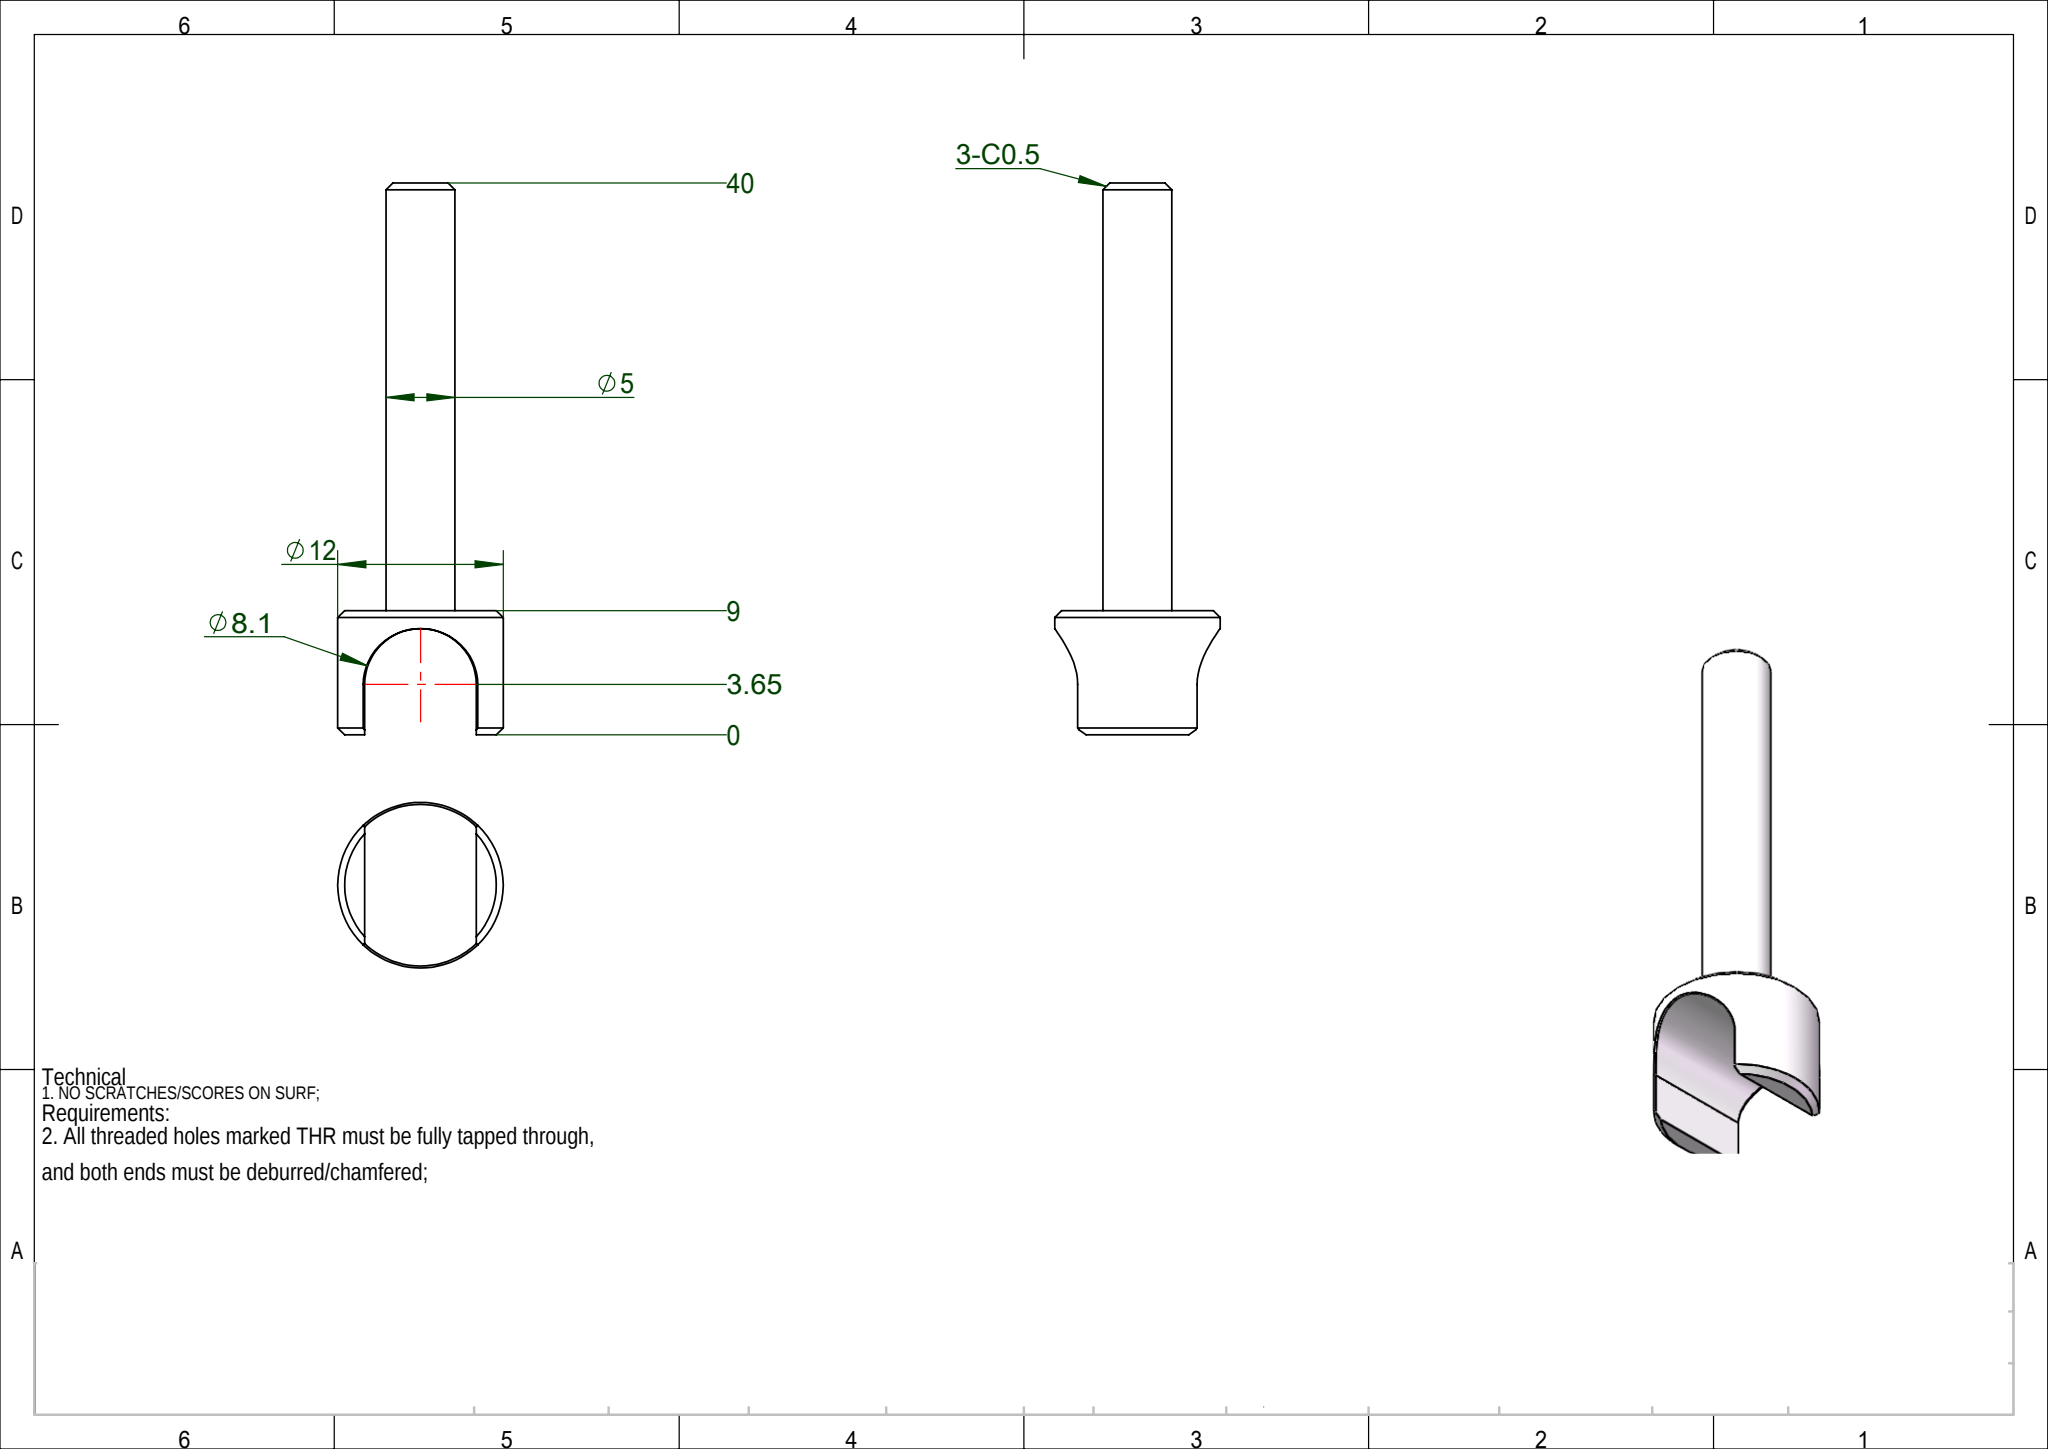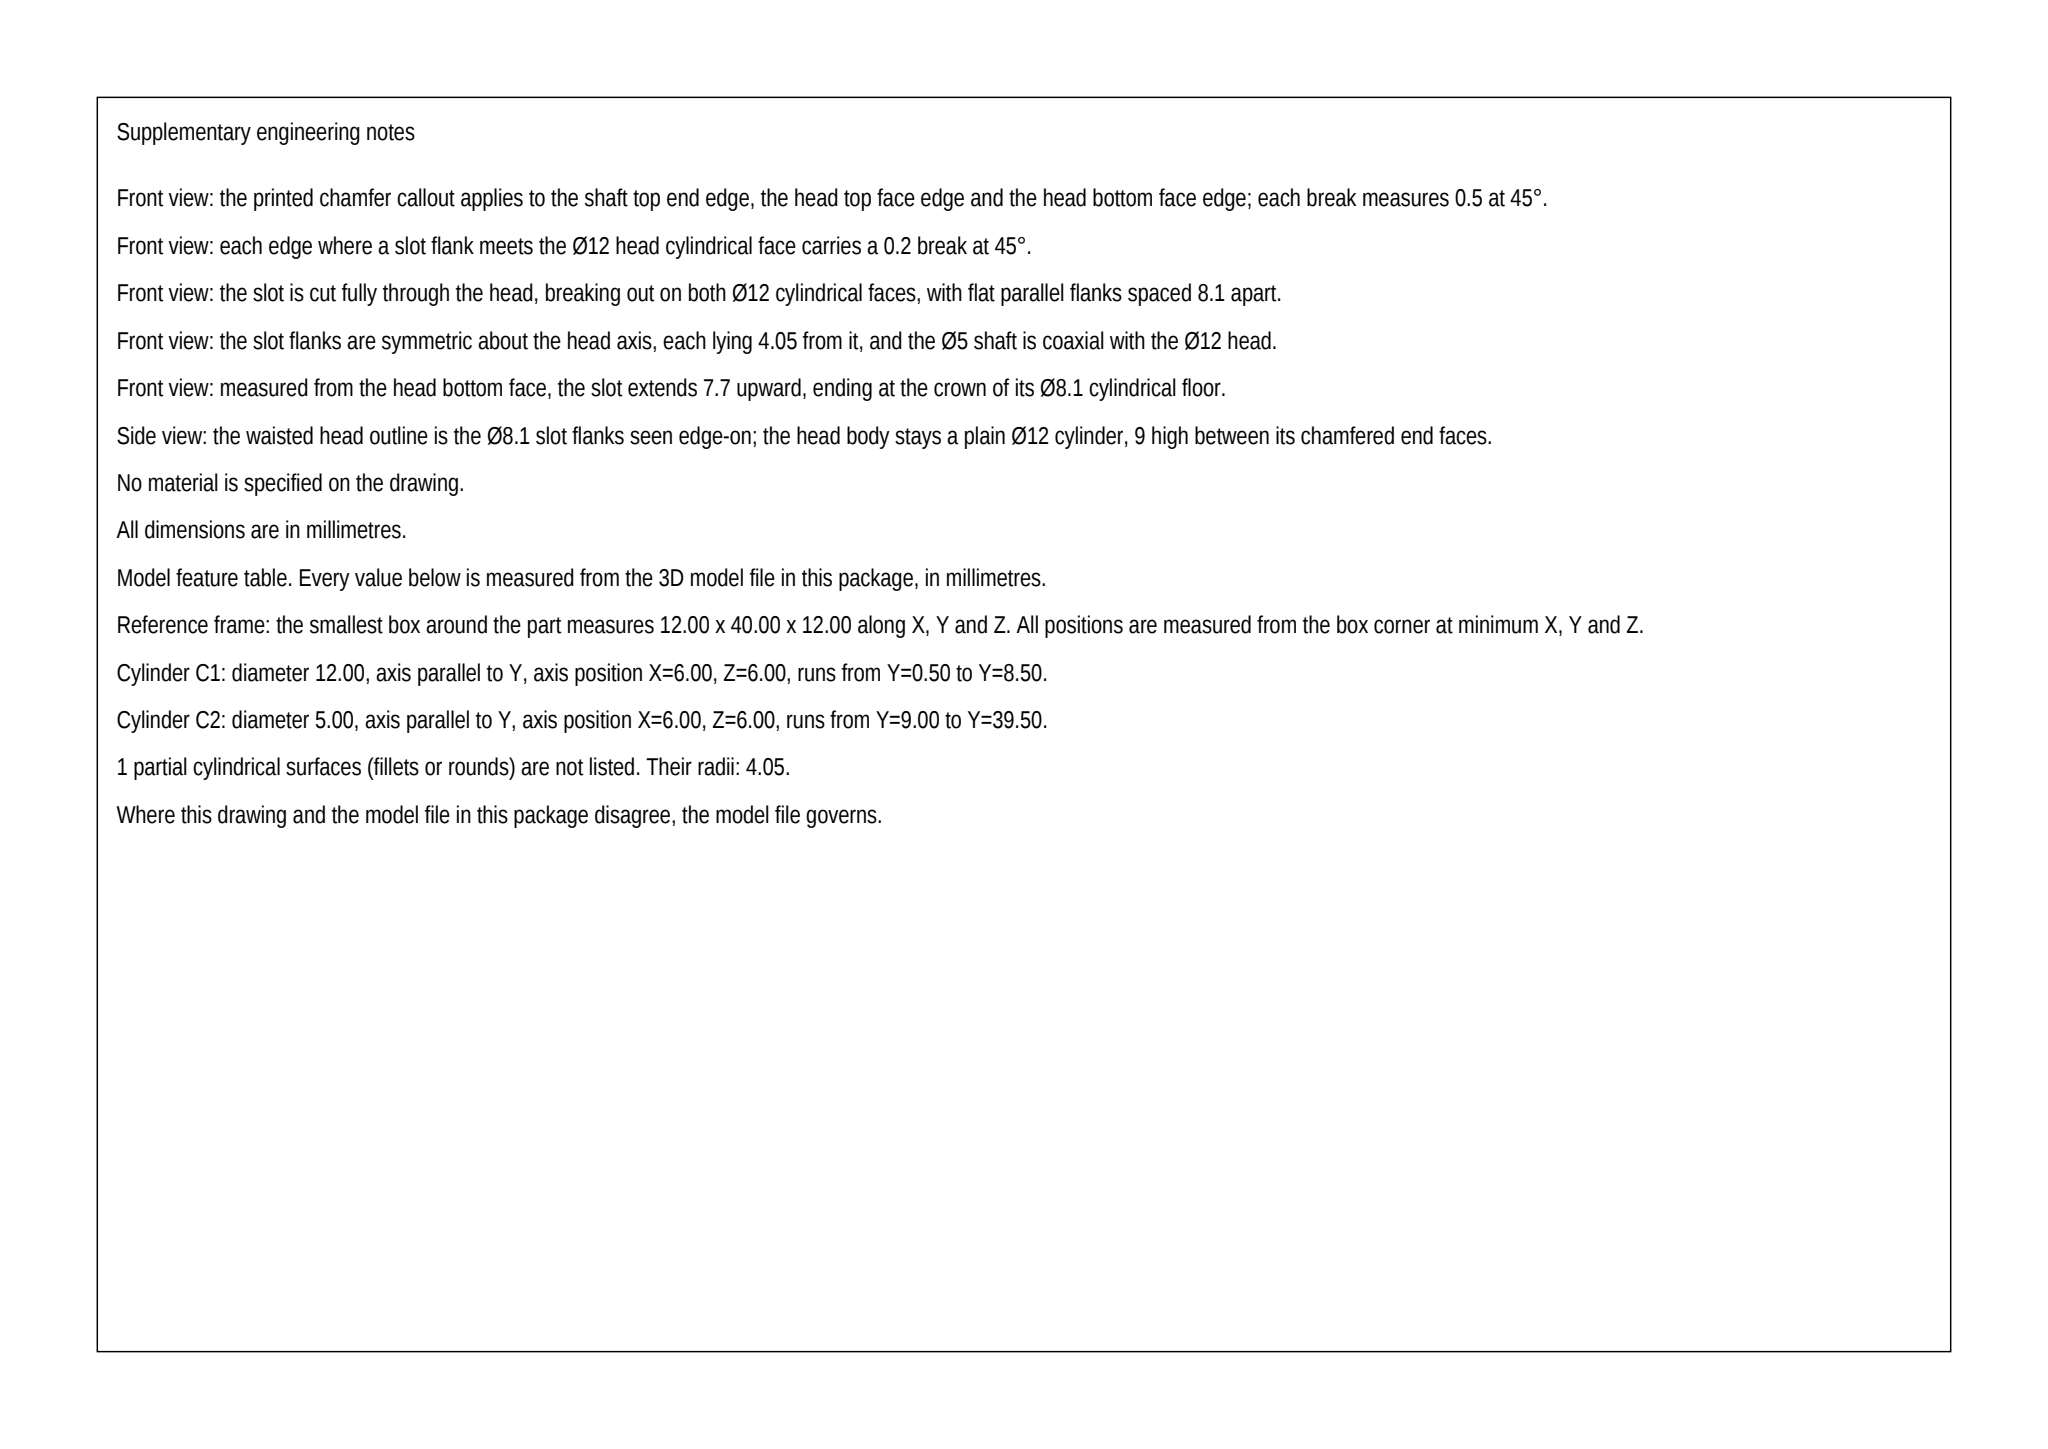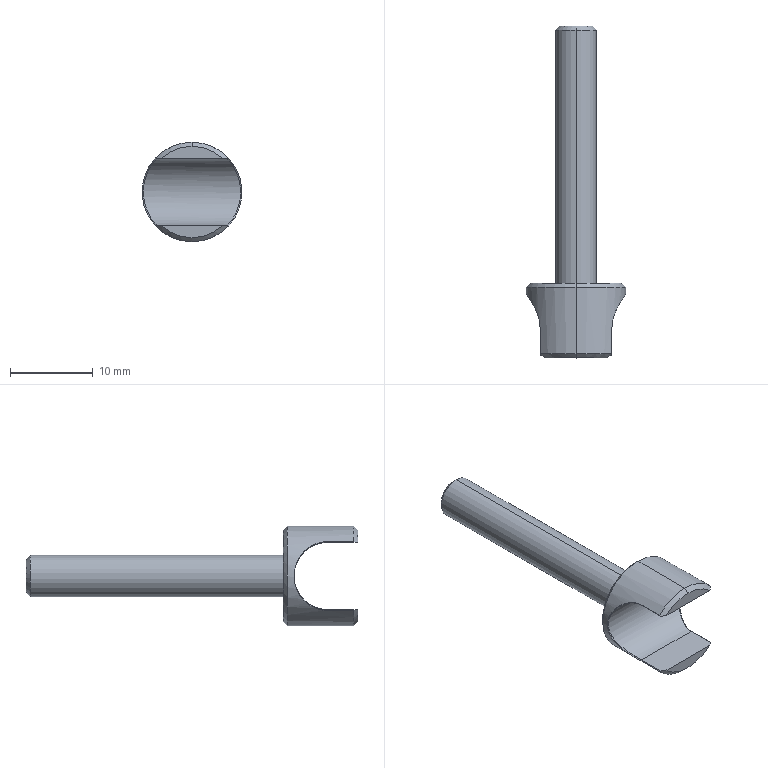Part | SolidWorks | mm | 1 solid | 24 faces | box 12 x 40 x 12 mm | volume 1001 mm3 | plane 10 | cone 7 | cylinder 5 | spline 2 | commonest cylinder face diameters 5 x2 12 x2 8.1 x1